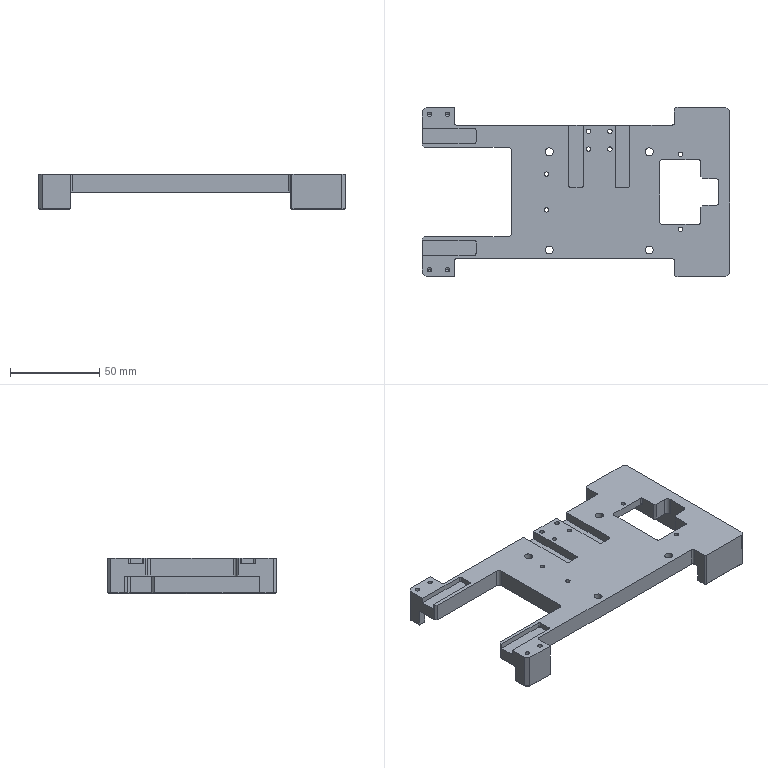Component | SolidWorks | Jig-1 | 1 solid | 218 faces | volume 103557 mm3 | plane 120 | cylinder 80 | cone 18 | commonest cylinder face diameters 2 x26 2.5 x24 4.5 x8 8 x8 4 x8 3.3 x4 6 x2